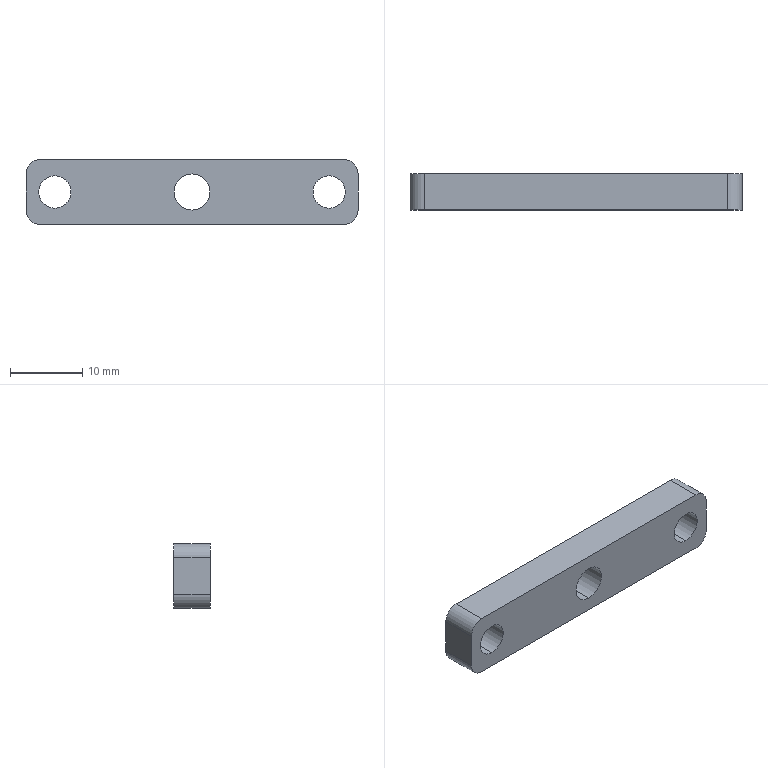Component | SolidWorks | 18ZTJ-NVT-01-011-1 | 1 solid | 16 faces | box 46 x 5 x 9 mm | volume 1796 mm3 | cylinder 10 | plane 6 | commonest cylinder face diameters 4.5 x4 4 x4 5 x2 | material #45
build123d program:
from build123d import *

# Parameters (mm, degrees)
SKETCH1_W                      = 46
SKETCH1_H                      = 9
BOSS_EXTRUDE1_DEPTH            = 5
M5_TAPPED_HOLE1_D              = 5
F_4_5_4_5_DIAMETER_HOLE1_D     = 4.5
F_4_5_4_5_DIAMETER_HOLE1_DEPTH = 10
F_4_5_4_5_DIAMETER_HOLE1_TIP   = 1.352
FILLET5_R                      = 2


with BuildPart() as part:
    # Sketch1 → Boss-Extrude1 (new body)
    with BuildSketch(Plane(origin=(0, 0, 0), x_dir=(1, 0, 0), z_dir=(0, 1, 0))):
        with Locations((23, 4.5)):
            Rectangle(SKETCH1_W, SKETCH1_H)
    extrude(amount=BOSS_EXTRUDE1_DEPTH)

    # M5 Tapped Hole1 (through all)
    with Locations(Plane(origin=(0, 5, 0), x_dir=(1, 0, 0), z_dir=(0, 1, 0))):
        with Locations((23, 4.5)):
            Hole(M5_TAPPED_HOLE1_D / 2)

    # 4.5 _4.5_ Diameter Hole1
    with Locations(Plane(origin=(0, 5, 0), x_dir=(1, 0, 0), z_dir=(0, 1, 0))):
        with Locations((42, 4.5), (4, 4.5)):
            Hole(F_4_5_4_5_DIAMETER_HOLE1_D / 2, depth=F_4_5_4_5_DIAMETER_HOLE1_DEPTH)
            with Locations((0, 0, -(F_4_5_4_5_DIAMETER_HOLE1_DEPTH + F_4_5_4_5_DIAMETER_HOLE1_TIP / 2))):  # 118° drill point
                Cone(0, F_4_5_4_5_DIAMETER_HOLE1_D / 2, F_4_5_4_5_DIAMETER_HOLE1_TIP, mode=Mode.SUBTRACT)

    # Fillet5
    fillet5_edges = [part.edges().sort_by_distance(p)[0] for p in [
        (0, 2.5, -9),
        (46, 2.5, -9),
        (46, 2.5, 0),
        (0, 2.5, 0),
    ]]
    fillet(fillet5_edges, radius=FILLET5_R)


solid = part.part

# Placed as in the assembly
solid = solid.moved(Location((-36.6, 22.47, 83.5), (0, 0, 0)))
STEP:
#1=COLOUR_RGB('',0.7922,0.8196,0.9333);
#2=FILL_AREA_STYLE_COLOUR('',#1);
#3=FILL_AREA_STYLE('',(#2));
#4=SURFACE_STYLE_FILL_AREA(#3);
#5=SURFACE_SIDE_STYLE('',(#4));
#6=SURFACE_STYLE_USAGE(.BOTH.,#5);
#7=PRESENTATION_STYLE_ASSIGNMENT((#6));
#8=CARTESIAN_POINT('',(0.2126,0.8847,3.199));
#9=VERTEX_POINT('',#8);
#10=CARTESIAN_POINT('',(0.2126,0.8847,3.022));
#11=VERTEX_POINT('',#10);
#12=CARTESIAN_POINT('',(0.2126,0.8847,3.11));
#13=DIRECTION('',(0.,-1.,0.));
#14=DIRECTION('',(0.,0.,-1.));
#15=AXIS2_PLACEMENT_3D('',#12,#13,#14);
#16=CIRCLE('',#15,0.08858);
#17=EDGE_CURVE('',#9,#11,#16,.T.);
#18=ORIENTED_EDGE('',*,*,#17,.T.);
#19=CARTESIAN_POINT('',(0.2126,1.082,3.022));
#20=VERTEX_POINT('',#19);
#21=CARTESIAN_POINT('',(0.2126,1.082,3.022));
#22=DIRECTION('',(0.,1.,0.));
#23=VECTOR('',#22,39.37);
#24=LINE('',#21,#23);
#25=EDGE_CURVE('',#11,#20,#24,.T.);
#26=ORIENTED_EDGE('',*,*,#25,.T.);
#27=CARTESIAN_POINT('',(0.2126,1.082,3.199));
#28=VERTEX_POINT('',#27);
#29=CARTESIAN_POINT('',(0.2126,1.082,3.11));
#30=DIRECTION('',(0.,1.,0.));
#31=DIRECTION('',(0.,0.,1.));
#32=AXIS2_PLACEMENT_3D('',#29,#30,#31);
#33=CIRCLE('',#32,0.08858);
#34=EDGE_CURVE('',#20,#28,#33,.T.);
#35=ORIENTED_EDGE('',*,*,#34,.T.);
#36=CARTESIAN_POINT('',(0.2126,1.082,3.199));
#37=DIRECTION('',(0.,1.,0.));
#38=VECTOR('',#37,39.37);
#39=LINE('',#36,#38);
#40=EDGE_CURVE('',#9,#28,#39,.T.);
#41=ORIENTED_EDGE('',*,*,#40,.F.);
#42=EDGE_LOOP('',(#18,#26,#35,#41));
#43=FACE_OUTER_BOUND('',#42,.T.);
#44=CARTESIAN_POINT('',(0.2126,1.082,3.11));
#45=DIRECTION('',(0.,1.,0.));
#46=DIRECTION('',(0.,0.,1.));
#47=AXIS2_PLACEMENT_3D('',#44,#45,#46);
#48=CYLINDRICAL_SURFACE('',#47,0.08858);
#49=ADVANCED_FACE('',(#43),#48,.F.);
#50=CARTESIAN_POINT('',(-1.283,0.8847,3.199));
#51=VERTEX_POINT('',#50);
#52=CARTESIAN_POINT('',(-1.283,0.8847,3.022));
#53=VERTEX_POINT('',#52);
#54=CARTESIAN_POINT('',(-1.283,0.8847,3.11));
#55=DIRECTION('',(0.,-1.,0.));
#56=DIRECTION('',(0.,0.,-1.));
#57=AXIS2_PLACEMENT_3D('',#54,#55,#56);
#58=CIRCLE('',#57,0.08858);
#59=EDGE_CURVE('',#51,#53,#58,.T.);
#60=ORIENTED_EDGE('',*,*,#59,.T.);
#61=CARTESIAN_POINT('',(-1.283,1.082,3.022));
#62=VERTEX_POINT('',#61);
#63=CARTESIAN_POINT('',(-1.283,1.082,3.022));
#64=DIRECTION('',(0.,1.,0.));
#65=VECTOR('',#64,39.37);
#66=LINE('',#63,#65);
#67=EDGE_CURVE('',#53,#62,#66,.T.);
#68=ORIENTED_EDGE('',*,*,#67,.T.);
#69=CARTESIAN_POINT('',(-1.283,1.082,3.199));
#70=VERTEX_POINT('',#69);
#71=CARTESIAN_POINT('',(-1.283,1.082,3.11));
#72=DIRECTION('',(0.,1.,0.));
#73=DIRECTION('',(0.,0.,1.));
#74=AXIS2_PLACEMENT_3D('',#71,#72,#73);
#75=CIRCLE('',#74,0.08858);
#76=EDGE_CURVE('',#62,#70,#75,.T.);
#77=ORIENTED_EDGE('',*,*,#76,.T.);
#78=CARTESIAN_POINT('',(-1.283,1.082,3.199));
#79=DIRECTION('',(0.,1.,0.));
#80=VECTOR('',#79,39.37);
#81=LINE('',#78,#80);
#82=EDGE_CURVE('',#51,#70,#81,.T.);
#83=ORIENTED_EDGE('',*,*,#82,.F.);
#84=EDGE_LOOP('',(#60,#68,#77,#83));
#85=FACE_OUTER_BOUND('',#84,.T.);
#86=CARTESIAN_POINT('',(-1.283,1.082,3.11));
#87=DIRECTION('',(0.,1.,0.));
#88=DIRECTION('',(0.,0.,1.));
#89=AXIS2_PLACEMENT_3D('',#86,#87,#88);
#90=CYLINDRICAL_SURFACE('',#89,0.08858);
#91=ADVANCED_FACE('',(#85),#90,.F.);
#92=CARTESIAN_POINT('',(-0.5354,0.8847,3.012));
#93=VERTEX_POINT('',#92);
#94=CARTESIAN_POINT('',(-0.5354,0.8847,3.209));
#95=VERTEX_POINT('',#94);
#96=CARTESIAN_POINT('',(-0.5354,0.8847,3.11));
#97=DIRECTION('',(0.,1.,0.));
#98=DIRECTION('',(0.,0.,1.));
#99=AXIS2_PLACEMENT_3D('',#96,#97,#98);
#100=CIRCLE('',#99,0.09843);
#101=EDGE_CURVE('',#93,#95,#100,.T.);
#102=ORIENTED_EDGE('',*,*,#101,.F.);
#103=CARTESIAN_POINT('',(-0.5354,1.082,3.012));
#104=VERTEX_POINT('',#103);
#105=CARTESIAN_POINT('',(-0.5354,1.082,3.012));
#106=DIRECTION('',(0.,1.,0.));
#107=VECTOR('',#106,39.37);
#108=LINE('',#105,#107);
#109=EDGE_CURVE('',#93,#104,#108,.T.);
#110=ORIENTED_EDGE('',*,*,#109,.T.);
#111=CARTESIAN_POINT('',(-0.5354,1.082,3.209));
#112=VERTEX_POINT('',#111);
#113=CARTESIAN_POINT('',(-0.5354,1.082,3.11));
#114=DIRECTION('',(0.,1.,0.));
#115=DIRECTION('',(0.,0.,1.));
#116=AXIS2_PLACEMENT_3D('',#113,#114,#115);
#117=CIRCLE('',#116,0.09843);
#118=EDGE_CURVE('',#104,#112,#117,.T.);
#119=ORIENTED_EDGE('',*,*,#118,.T.);
#120=CARTESIAN_POINT('',(-0.5354,1.082,3.209));
#121=DIRECTION('',(0.,1.,0.));
#122=VECTOR('',#121,39.37);
#123=LINE('',#120,#122);
#124=EDGE_CURVE('',#95,#112,#123,.T.);
#125=ORIENTED_EDGE('',*,*,#124,.F.);
#126=EDGE_LOOP('',(#102,#110,#119,#125));
#127=FACE_OUTER_BOUND('',#126,.T.);
#128=CARTESIAN_POINT('',(-0.5354,1.082,3.11));
#129=DIRECTION('',(0.,1.,0.));
#130=DIRECTION('',(0.,0.,1.));
#131=AXIS2_PLACEMENT_3D('',#128,#129,#130);
#132=CYLINDRICAL_SURFACE('',#131,0.09843);
#133=ADVANCED_FACE('',(#127),#132,.F.);
#134=ORIENTED_EDGE('',*,*,#17,.F.);
#135=CARTESIAN_POINT('',(0.2126,0.8847,3.11));
#136=DIRECTION('',(0.,-1.,0.));
#137=DIRECTION('',(0.,0.,-1.));
#138=AXIS2_PLACEMENT_3D('',#135,#136,#137);
#139=CIRCLE('',#138,0.08858);
#140=EDGE_CURVE('',#11,#9,#139,.T.);
#141=ORIENTED_EDGE('',*,*,#140,.F.);
#142=EDGE_LOOP('',(#134,#141));
#143=FACE_BOUND('',#142,.T.);
#144=ORIENTED_EDGE('',*,*,#59,.F.);
#145=CARTESIAN_POINT('',(-1.283,0.8847,3.11));
#146=DIRECTION('',(0.,-1.,0.));
#147=DIRECTION('',(0.,0.,-1.));
#148=AXIS2_PLACEMENT_3D('',#145,#146,#147);
#149=CIRCLE('',#148,0.08858);
#150=EDGE_CURVE('',#53,#51,#149,.T.);
#151=ORIENTED_EDGE('',*,*,#150,.F.);
#152=EDGE_LOOP('',(#144,#151));
#153=FACE_BOUND('',#152,.T.);
#154=CARTESIAN_POINT('',(-1.441,0.8847,3.012));
#155=VERTEX_POINT('',#154);
#156=CARTESIAN_POINT('',(-1.441,0.8847,3.209));
#157=VERTEX_POINT('',#156);
#158=CARTESIAN_POINT('',(-1.441,0.8847,3.287));
#159=DIRECTION('',(0.,0.,1.));
#160=VECTOR('',#159,39.37);
#161=LINE('',#158,#160);
#162=EDGE_CURVE('',#155,#157,#161,.T.);
#163=ORIENTED_EDGE('',*,*,#162,.F.);
#164=CARTESIAN_POINT('',(-1.362,0.8847,2.933));
#165=VERTEX_POINT('',#164);
#166=CARTESIAN_POINT('',(-1.362,0.8847,3.012));
#167=DIRECTION('',(0.,-1.,0.));
#168=DIRECTION('',(0.,0.,-1.));
#169=AXIS2_PLACEMENT_3D('',#166,#167,#168);
#170=CIRCLE('',#169,0.07874);
#171=EDGE_CURVE('',#155,#165,#170,.T.);
#172=ORIENTED_EDGE('',*,*,#171,.T.);
#173=CARTESIAN_POINT('',(0.2914,0.8847,2.933));
#174=VERTEX_POINT('',#173);
#175=CARTESIAN_POINT('',(-1.441,0.8847,2.933));
#176=DIRECTION('',(-1.,0.,0.));
#177=VECTOR('',#176,39.37);
#178=LINE('',#175,#177);
#179=EDGE_CURVE('',#174,#165,#178,.T.);
#180=ORIENTED_EDGE('',*,*,#179,.F.);
#181=CARTESIAN_POINT('',(0.3701,0.8847,3.012));
#182=VERTEX_POINT('',#181);
#183=CARTESIAN_POINT('',(0.2914,0.8847,3.012));
#184=DIRECTION('',(0.,-1.,0.));
#185=DIRECTION('',(0.,0.,-1.));
#186=AXIS2_PLACEMENT_3D('',#183,#184,#185);
#187=CIRCLE('',#186,0.07874);
#188=EDGE_CURVE('',#174,#182,#187,.T.);
#189=ORIENTED_EDGE('',*,*,#188,.T.);
#190=CARTESIAN_POINT('',(0.3701,0.8847,3.209));
#191=VERTEX_POINT('',#190);
#192=CARTESIAN_POINT('',(0.3701,0.8847,3.287));
#193=DIRECTION('',(0.,0.,-1.));
#194=VECTOR('',#193,39.37);
#195=LINE('',#192,#194);
#196=EDGE_CURVE('',#191,#182,#195,.T.);
#197=ORIENTED_EDGE('',*,*,#196,.F.);
#198=CARTESIAN_POINT('',(0.2914,0.8847,3.287));
#199=VERTEX_POINT('',#198);
#200=CARTESIAN_POINT('',(0.2914,0.8847,3.209));
#201=DIRECTION('',(0.,-1.,0.));
#202=DIRECTION('',(0.,0.,-1.));
#203=AXIS2_PLACEMENT_3D('',#200,#201,#202);
#204=CIRCLE('',#203,0.07874);
#205=EDGE_CURVE('',#191,#199,#204,.T.);
#206=ORIENTED_EDGE('',*,*,#205,.T.);
#207=CARTESIAN_POINT('',(-1.362,0.8847,3.287));
#208=VERTEX_POINT('',#207);
#209=CARTESIAN_POINT('',(-1.441,0.8847,3.287));
#210=DIRECTION('',(1.,0.,0.));
#211=VECTOR('',#210,39.37);
#212=LINE('',#209,#211);
#213=EDGE_CURVE('',#208,#199,#212,.T.);
#214=ORIENTED_EDGE('',*,*,#213,.F.);
#215=CARTESIAN_POINT('',(-1.362,0.8847,3.209));
#216=DIRECTION('',(0.,-1.,0.));
#217=DIRECTION('',(0.,0.,-1.));
#218=AXIS2_PLACEMENT_3D('',#215,#216,#217);
#219=CIRCLE('',#218,0.07874);
#220=EDGE_CURVE('',#208,#157,#219,.T.);
#221=ORIENTED_EDGE('',*,*,#220,.T.);
#222=EDGE_LOOP('',(#163,#172,#180,#189,#197,#206,#214,#221));
#223=FACE_OUTER_BOUND('',#222,.T.);
#224=CARTESIAN_POINT('',(-0.5354,0.8847,3.11));
#225=DIRECTION('',(0.,1.,0.));
#226=DIRECTION('',(0.,0.,1.));
#227=AXIS2_PLACEMENT_3D('',#224,#225,#226);
#228=CIRCLE('',#227,0.09843);
#229=EDGE_CURVE('',#95,#93,#228,.T.);
#230=ORIENTED_EDGE('',*,*,#229,.T.);
#231=ORIENTED_EDGE('',*,*,#101,.T.);
#232=EDGE_LOOP('',(#230,#231));
#233=FACE_BOUND('',#232,.T.);
#234=CARTESIAN_POINT('',(-1.441,0.8847,3.287));
#235=DIRECTION('',(0.,-1.,0.));
#236=DIRECTION('',(0.,0.,-1.));
#237=AXIS2_PLACEMENT_3D('',#234,#235,#236);
#238=PLANE('',#237);
#239=ADVANCED_FACE('',(#143,#153,#223,#233),#238,.T.);
#240=CARTESIAN_POINT('',(-1.441,1.082,3.012));
#241=VERTEX_POINT('',#240);
#242=CARTESIAN_POINT('',(-1.441,1.082,3.209));
#243=VERTEX_POINT('',#242);
#244=CARTESIAN_POINT('',(-1.441,1.082,3.287));
#245=DIRECTION('',(0.,0.,1.));
#246=VECTOR('',#245,39.37);
#247=LINE('',#244,#246);
#248=EDGE_CURVE('',#241,#243,#247,.T.);
#249=ORIENTED_EDGE('',*,*,#248,.F.);
#250=CARTESIAN_POINT('',(-1.441,1.082,3.012));
#251=DIRECTION('',(0.,-1.,0.));
#252=VECTOR('',#251,39.37);
#253=LINE('',#250,#252);
#254=EDGE_CURVE('',#241,#155,#253,.T.);
#255=ORIENTED_EDGE('',*,*,#254,.T.);
#256=ORIENTED_EDGE('',*,*,#162,.T.);
#257=CARTESIAN_POINT('',(-1.441,1.082,3.209));
#258=DIRECTION('',(0.,1.,0.));
#259=VECTOR('',#258,39.37);
#260=LINE('',#257,#259);
#261=EDGE_CURVE('',#157,#243,#260,.T.);
#262=ORIENTED_EDGE('',*,*,#261,.T.);
#263=EDGE_LOOP('',(#249,#255,#256,#262));
#264=FACE_OUTER_BOUND('',#263,.T.);
#265=CARTESIAN_POINT('',(-1.441,1.082,3.287));
#266=DIRECTION('',(1.,0.,0.));
#267=DIRECTION('',(0.,0.,-1.));
#268=AXIS2_PLACEMENT_3D('',#265,#266,#267);
#269=PLANE('',#268);
#270=ADVANCED_FACE('',(#264),#269,.F.);
#271=CARTESIAN_POINT('',(-1.362,1.082,3.287));
#272=VERTEX_POINT('',#271);
#273=CARTESIAN_POINT('',(0.2914,1.082,3.287));
#274=VERTEX_POINT('',#273);
#275=CARTESIAN_POINT('',(-1.441,1.082,3.287));
#276=DIRECTION('',(1.,0.,0.));
#277=VECTOR('',#276,39.37);
#278=LINE('',#275,#277);
#279=EDGE_CURVE('',#272,#274,#278,.T.);
#280=ORIENTED_EDGE('',*,*,#279,.F.);
#281=CARTESIAN_POINT('',(-1.362,1.082,3.287));
#282=DIRECTION('',(0.,-1.,0.));
#283=VECTOR('',#282,39.37);
#284=LINE('',#281,#283);
#285=EDGE_CURVE('',#272,#208,#284,.T.);
#286=ORIENTED_EDGE('',*,*,#285,.T.);
#287=ORIENTED_EDGE('',*,*,#213,.T.);
#288=CARTESIAN_POINT('',(0.2914,1.082,3.287));
#289=DIRECTION('',(0.,1.,0.));
#290=VECTOR('',#289,39.37);
#291=LINE('',#288,#290);
#292=EDGE_CURVE('',#199,#274,#291,.T.);
#293=ORIENTED_EDGE('',*,*,#292,.T.);
#294=EDGE_LOOP('',(#280,#286,#287,#293));
#295=FACE_OUTER_BOUND('',#294,.T.);
#296=CARTESIAN_POINT('',(-1.441,1.082,3.287));
#297=DIRECTION('',(0.,0.,-1.));
#298=DIRECTION('',(-1.,0.,0.));
#299=AXIS2_PLACEMENT_3D('',#296,#297,#298);
#300=PLANE('',#299);
#301=ADVANCED_FACE('',(#295),#300,.F.);
#302=ORIENTED_EDGE('',*,*,#196,.T.);
#303=CARTESIAN_POINT('',(0.3701,1.082,3.012));
#304=VERTEX_POINT('',#303);
#305=CARTESIAN_POINT('',(0.3701,1.082,3.012));
#306=DIRECTION('',(0.,1.,0.));
#307=VECTOR('',#306,39.37);
#308=LINE('',#305,#307);
#309=EDGE_CURVE('',#182,#304,#308,.T.);
#310=ORIENTED_EDGE('',*,*,#309,.T.);
#311=CARTESIAN_POINT('',(0.3701,1.082,3.209));
#312=VERTEX_POINT('',#311);
#313=CARTESIAN_POINT('',(0.3701,1.082,3.287));
#314=DIRECTION('',(0.,0.,-1.));
#315=VECTOR('',#314,39.37);
#316=LINE('',#313,#315);
#317=EDGE_CURVE('',#312,#304,#316,.T.);
#318=ORIENTED_EDGE('',*,*,#317,.F.);
#319=CARTESIAN_POINT('',(0.3701,1.082,3.209));
#320=DIRECTION('',(0.,-1.,0.));
#321=VECTOR('',#320,39.37);
#322=LINE('',#319,#321);
#323=EDGE_CURVE('',#312,#191,#322,.T.);
#324=ORIENTED_EDGE('',*,*,#323,.T.);
#325=EDGE_LOOP('',(#302,#310,#318,#324));
#326=FACE_OUTER_BOUND('',#325,.T.);
#327=CARTESIAN_POINT('',(0.3701,1.082,3.287));
#328=DIRECTION('',(-1.,0.,0.));
#329=DIRECTION('',(0.,0.,1.));
#330=AXIS2_PLACEMENT_3D('',#327,#328,#329);
#331=PLANE('',#330);
#332=ADVANCED_FACE('',(#326),#331,.F.);
#333=ORIENTED_EDGE('',*,*,#179,.T.);
#334=CARTESIAN_POINT('',(-1.362,1.082,2.933));
#335=VERTEX_POINT('',#334);
#336=CARTESIAN_POINT('',(-1.362,1.082,2.933));
#337=DIRECTION('',(0.,1.,0.));
#338=VECTOR('',#337,39.37);
#339=LINE('',#336,#338);
#340=EDGE_CURVE('',#165,#335,#339,.T.);
#341=ORIENTED_EDGE('',*,*,#340,.T.);
#342=CARTESIAN_POINT('',(0.2914,1.082,2.933));
#343=VERTEX_POINT('',#342);
#344=CARTESIAN_POINT('',(-1.441,1.082,2.933));
#345=DIRECTION('',(-1.,0.,0.));
#346=VECTOR('',#345,39.37);
#347=LINE('',#344,#346);
#348=EDGE_CURVE('',#343,#335,#347,.T.);
#349=ORIENTED_EDGE('',*,*,#348,.F.);
#350=CARTESIAN_POINT('',(0.2914,1.082,2.933));
#351=DIRECTION('',(0.,-1.,0.));
#352=VECTOR('',#351,39.37);
#353=LINE('',#350,#352);
#354=EDGE_CURVE('',#343,#174,#353,.T.);
#355=ORIENTED_EDGE('',*,*,#354,.T.);
#356=EDGE_LOOP('',(#333,#341,#349,#355));
#357=FACE_OUTER_BOUND('',#356,.T.);
#358=CARTESIAN_POINT('',(-1.441,1.082,2.933));
#359=DIRECTION('',(0.,0.,1.));
#360=DIRECTION('',(1.,0.,0.));
#361=AXIS2_PLACEMENT_3D('',#358,#359,#360);
#362=PLANE('',#361);
#363=ADVANCED_FACE('',(#357),#362,.F.);
#364=CARTESIAN_POINT('',(0.2126,1.082,3.11));
#365=DIRECTION('',(0.,1.,0.));
#366=DIRECTION('',(0.,0.,1.));
#367=AXIS2_PLACEMENT_3D('',#364,#365,#366);
#368=CIRCLE('',#367,0.08858);
#369=EDGE_CURVE('',#28,#20,#368,.T.);
#370=ORIENTED_EDGE('',*,*,#369,.F.);
#371=ORIENTED_EDGE('',*,*,#34,.F.);
#372=EDGE_LOOP('',(#370,#371));
#373=FACE_BOUND('',#372,.T.);
#374=CARTESIAN_POINT('',(-1.283,1.082,3.11));
#375=DIRECTION('',(0.,1.,0.));
#376=DIRECTION('',(0.,0.,1.));
#377=AXIS2_PLACEMENT_3D('',#374,#375,#376);
#378=CIRCLE('',#377,0.08858);
#379=EDGE_CURVE('',#70,#62,#378,.T.);
#380=ORIENTED_EDGE('',*,*,#379,.F.);
#381=ORIENTED_EDGE('',*,*,#76,.F.);
#382=EDGE_LOOP('',(#380,#381));
#383=FACE_BOUND('',#382,.T.);
#384=CARTESIAN_POINT('',(-0.5354,1.082,3.11));
#385=DIRECTION('',(0.,1.,0.));
#386=DIRECTION('',(0.,0.,1.));
#387=AXIS2_PLACEMENT_3D('',#384,#385,#386);
#388=CIRCLE('',#387,0.09843);
#389=EDGE_CURVE('',#112,#104,#388,.T.);
#390=ORIENTED_EDGE('',*,*,#389,.F.);
#391=ORIENTED_EDGE('',*,*,#118,.F.);
#392=EDGE_LOOP('',(#390,#391));
#393=FACE_BOUND('',#392,.T.);
#394=ORIENTED_EDGE('',*,*,#348,.T.);
#395=CARTESIAN_POINT('',(-1.362,1.082,3.012));
#396=DIRECTION('',(0.,1.,0.));
#397=DIRECTION('',(0.,0.,-1.));
#398=AXIS2_PLACEMENT_3D('',#395,#396,#397);
#399=CIRCLE('',#398,0.07874);
#400=EDGE_CURVE('',#335,#241,#399,.T.);
#401=ORIENTED_EDGE('',*,*,#400,.T.);
#402=ORIENTED_EDGE('',*,*,#248,.T.);
#403=CARTESIAN_POINT('',(-1.362,1.082,3.209));
#404=DIRECTION('',(0.,1.,0.));
#405=DIRECTION('',(0.,0.,-1.));
#406=AXIS2_PLACEMENT_3D('',#403,#404,#405);
#407=CIRCLE('',#406,0.07874);
#408=EDGE_CURVE('',#243,#272,#407,.T.);
#409=ORIENTED_EDGE('',*,*,#408,.T.);
#410=ORIENTED_EDGE('',*,*,#279,.T.);
#411=CARTESIAN_POINT('',(0.2914,1.082,3.209));
#412=DIRECTION('',(0.,1.,0.));
#413=DIRECTION('',(0.,0.,-1.));
#414=AXIS2_PLACEMENT_3D('',#411,#412,#413);
#415=CIRCLE('',#414,0.07874);
#416=EDGE_CURVE('',#274,#312,#415,.T.);
#417=ORIENTED_EDGE('',*,*,#416,.T.);
#418=ORIENTED_EDGE('',*,*,#317,.T.);
#419=CARTESIAN_POINT('',(0.2914,1.082,3.012));
#420=DIRECTION('',(0.,1.,0.));
#421=DIRECTION('',(0.,0.,-1.));
#422=AXIS2_PLACEMENT_3D('',#419,#420,#421);
#423=CIRCLE('',#422,0.07874);
#424=EDGE_CURVE('',#304,#343,#423,.T.);
#425=ORIENTED_EDGE('',*,*,#424,.T.);
#426=EDGE_LOOP('',(#394,#401,#402,#409,#410,#417,#418,#425));
#427=FACE_OUTER_BOUND('',#426,.T.);
#428=CARTESIAN_POINT('',(-1.441,1.082,3.287));
#429=DIRECTION('',(0.,-1.,0.));
#430=DIRECTION('',(0.,0.,-1.));
#431=AXIS2_PLACEMENT_3D('',#428,#429,#430);
#432=PLANE('',#431);
#433=ADVANCED_FACE('',(#373,#383,#393,#427),#432,.F.);
#434=ORIENTED_EDGE('',*,*,#109,.F.);
#435=ORIENTED_EDGE('',*,*,#229,.F.);
#436=ORIENTED_EDGE('',*,*,#124,.T.);
#437=ORIENTED_EDGE('',*,*,#389,.T.);
#438=EDGE_LOOP('',(#434,#435,#436,#437));
#439=FACE_OUTER_BOUND('',#438,.T.);
#440=CARTESIAN_POINT('',(-0.5354,1.082,3.11));
#441=DIRECTION('',(0.,1.,0.));
#442=DIRECTION('',(0.,0.,1.));
#443=AXIS2_PLACEMENT_3D('',#440,#441,#442);
#444=CYLINDRICAL_SURFACE('',#443,0.09843);
#445=ADVANCED_FACE('',(#439),#444,.F.);
#446=ORIENTED_EDGE('',*,*,#67,.F.);
#447=ORIENTED_EDGE('',*,*,#150,.T.);
#448=ORIENTED_EDGE('',*,*,#82,.T.);
#449=ORIENTED_EDGE('',*,*,#379,.T.);
#450=EDGE_LOOP('',(#446,#447,#448,#449));
#451=FACE_OUTER_BOUND('',#450,.T.);
#452=CARTESIAN_POINT('',(-1.283,1.082,3.11));
#453=DIRECTION('',(0.,1.,0.));
#454=DIRECTION('',(0.,0.,1.));
#455=AXIS2_PLACEMENT_3D('',#452,#453,#454);
#456=CYLINDRICAL_SURFACE('',#455,0.08858);
#457=ADVANCED_FACE('',(#451),#456,.F.);
#458=ORIENTED_EDGE('',*,*,#25,.F.);
#459=ORIENTED_EDGE('',*,*,#140,.T.);
#460=ORIENTED_EDGE('',*,*,#40,.T.);
#461=ORIENTED_EDGE('',*,*,#369,.T.);
#462=EDGE_LOOP('',(#458,#459,#460,#461));
#463=FACE_OUTER_BOUND('',#462,.T.);
#464=CARTESIAN_POINT('',(0.2126,1.082,3.11));
#465=DIRECTION('',(0.,1.,0.));
#466=DIRECTION('',(0.,0.,1.));
#467=AXIS2_PLACEMENT_3D('',#464,#465,#466);
#468=CYLINDRICAL_SURFACE('',#467,0.08858);
#469=ADVANCED_FACE('',(#463),#468,.F.);
#470=ORIENTED_EDGE('',*,*,#400,.F.);
#471=ORIENTED_EDGE('',*,*,#340,.F.);
#472=ORIENTED_EDGE('',*,*,#171,.F.);
#473=ORIENTED_EDGE('',*,*,#254,.F.);
#474=EDGE_LOOP('',(#470,#471,#472,#473));
#475=FACE_OUTER_BOUND('',#474,.T.);
#476=CARTESIAN_POINT('',(-1.362,1.082,3.012));
#477=DIRECTION('',(0.,-1.,0.));
#478=DIRECTION('',(0.,0.,-1.));
#479=AXIS2_PLACEMENT_3D('',#476,#477,#478);
#480=CYLINDRICAL_SURFACE('',#479,0.07874);
#481=ADVANCED_FACE('',(#475),#480,.T.);
#482=ORIENTED_EDGE('',*,*,#408,.F.);
#483=ORIENTED_EDGE('',*,*,#261,.F.);
#484=ORIENTED_EDGE('',*,*,#220,.F.);
#485=ORIENTED_EDGE('',*,*,#285,.F.);
#486=EDGE_LOOP('',(#482,#483,#484,#485));
#487=FACE_OUTER_BOUND('',#486,.T.);
#488=CARTESIAN_POINT('',(-1.362,1.082,3.209));
#489=DIRECTION('',(0.,-1.,0.));
#490=DIRECTION('',(0.,0.,-1.));
#491=AXIS2_PLACEMENT_3D('',#488,#489,#490);
#492=CYLINDRICAL_SURFACE('',#491,0.07874);
#493=ADVANCED_FACE('',(#487),#492,.T.);
#494=ORIENTED_EDGE('',*,*,#424,.F.);
#495=ORIENTED_EDGE('',*,*,#309,.F.);
#496=ORIENTED_EDGE('',*,*,#188,.F.);
#497=ORIENTED_EDGE('',*,*,#354,.F.);
#498=EDGE_LOOP('',(#494,#495,#496,#497));
#499=FACE_OUTER_BOUND('',#498,.T.);
#500=CARTESIAN_POINT('',(0.2914,1.082,3.012));
#501=DIRECTION('',(0.,-1.,0.));
#502=DIRECTION('',(0.,0.,-1.));
#503=AXIS2_PLACEMENT_3D('',#500,#501,#502);
#504=CYLINDRICAL_SURFACE('',#503,0.07874);
#505=ADVANCED_FACE('',(#499),#504,.T.);
#506=ORIENTED_EDGE('',*,*,#416,.F.);
#507=ORIENTED_EDGE('',*,*,#292,.F.);
#508=ORIENTED_EDGE('',*,*,#205,.F.);
#509=ORIENTED_EDGE('',*,*,#323,.F.);
#510=EDGE_LOOP('',(#506,#507,#508,#509));
#511=FACE_OUTER_BOUND('',#510,.T.);
#512=CARTESIAN_POINT('',(0.2914,1.082,3.209));
#513=DIRECTION('',(0.,-1.,0.));
#514=DIRECTION('',(0.,0.,-1.));
#515=AXIS2_PLACEMENT_3D('',#512,#513,#514);
#516=CYLINDRICAL_SURFACE('',#515,0.07874);
#517=ADVANCED_FACE('',(#511),#516,.T.);
#518=CLOSED_SHELL('',(#49,#91,#133,#239,#270,#301,#332,#363,#433,#445,#457,#469,#481,#493,#505,#517));
#519=MANIFOLD_SOLID_BREP('',#518);
#520=STYLED_ITEM('',(#7),#519);
#521=PRESENTATION_LAYER_ASSIGNMENT('','',(#520));
#522=CARTESIAN_POINT('',(0.,0.,0.));
#523=DIRECTION('',(0.,0.,1.));
#524=DIRECTION('',(1.,0.,0.));
#525=AXIS2_PLACEMENT_3D('',#522,#523,#524);
#526=(LENGTH_UNIT()NAMED_UNIT(*)SI_UNIT($,.METRE.));
#527=LENGTH_MEASURE_WITH_UNIT(LENGTH_MEASURE(0.0254),#526);
#528=DIMENSIONAL_EXPONENTS(1.,0.,0.,0.,0.,0.,0.);
#529=(CONVERSION_BASED_UNIT('',#527)LENGTH_UNIT()NAMED_UNIT(#528));
#530=UNCERTAINTY_MEASURE_WITH_UNIT(LENGTH_MEASURE(0.00001),#529,'','');
#531=(NAMED_UNIT(*)PLANE_ANGLE_UNIT()SI_UNIT($,.RADIAN.));
#532=(NAMED_UNIT(*)SI_UNIT($,.STERADIAN.)SOLID_ANGLE_UNIT());
#533=(GEOMETRIC_REPRESENTATION_CONTEXT(3)GLOBAL_UNCERTAINTY_ASSIGNED_CONTEXT((#530))GLOBAL_UNIT_ASSIGNED_CONTEXT((#529,#531,#532))REPRESENTATION_CONTEXT('',''));
#534=ADVANCED_BREP_SHAPE_REPRESENTATION('',(#519,#525),#533);
#535=(LENGTH_UNIT()NAMED_UNIT(*)SI_UNIT($,.METRE.));
#536=LENGTH_MEASURE_WITH_UNIT(LENGTH_MEASURE(0.0254),#535);
#537=DIMENSIONAL_EXPONENTS(1.,0.,0.,0.,0.,0.,0.);
#538=(CONVERSION_BASED_UNIT('',#536)LENGTH_UNIT()NAMED_UNIT(#537));
#539=UNCERTAINTY_MEASURE_WITH_UNIT(LENGTH_MEASURE(0.00001),#538,'','');
#540=(NAMED_UNIT(*)PLANE_ANGLE_UNIT()SI_UNIT($,.RADIAN.));
#541=(NAMED_UNIT(*)SI_UNIT($,.STERADIAN.)SOLID_ANGLE_UNIT());
#542=(GEOMETRIC_REPRESENTATION_CONTEXT(3)GLOBAL_UNCERTAINTY_ASSIGNED_CONTEXT((#539))GLOBAL_UNIT_ASSIGNED_CONTEXT((#538,#540,#541))REPRESENTATION_CONTEXT('',''));
#543=MECHANICAL_DESIGN_GEOMETRIC_PRESENTATION_REPRESENTATION('',(#520),#542);